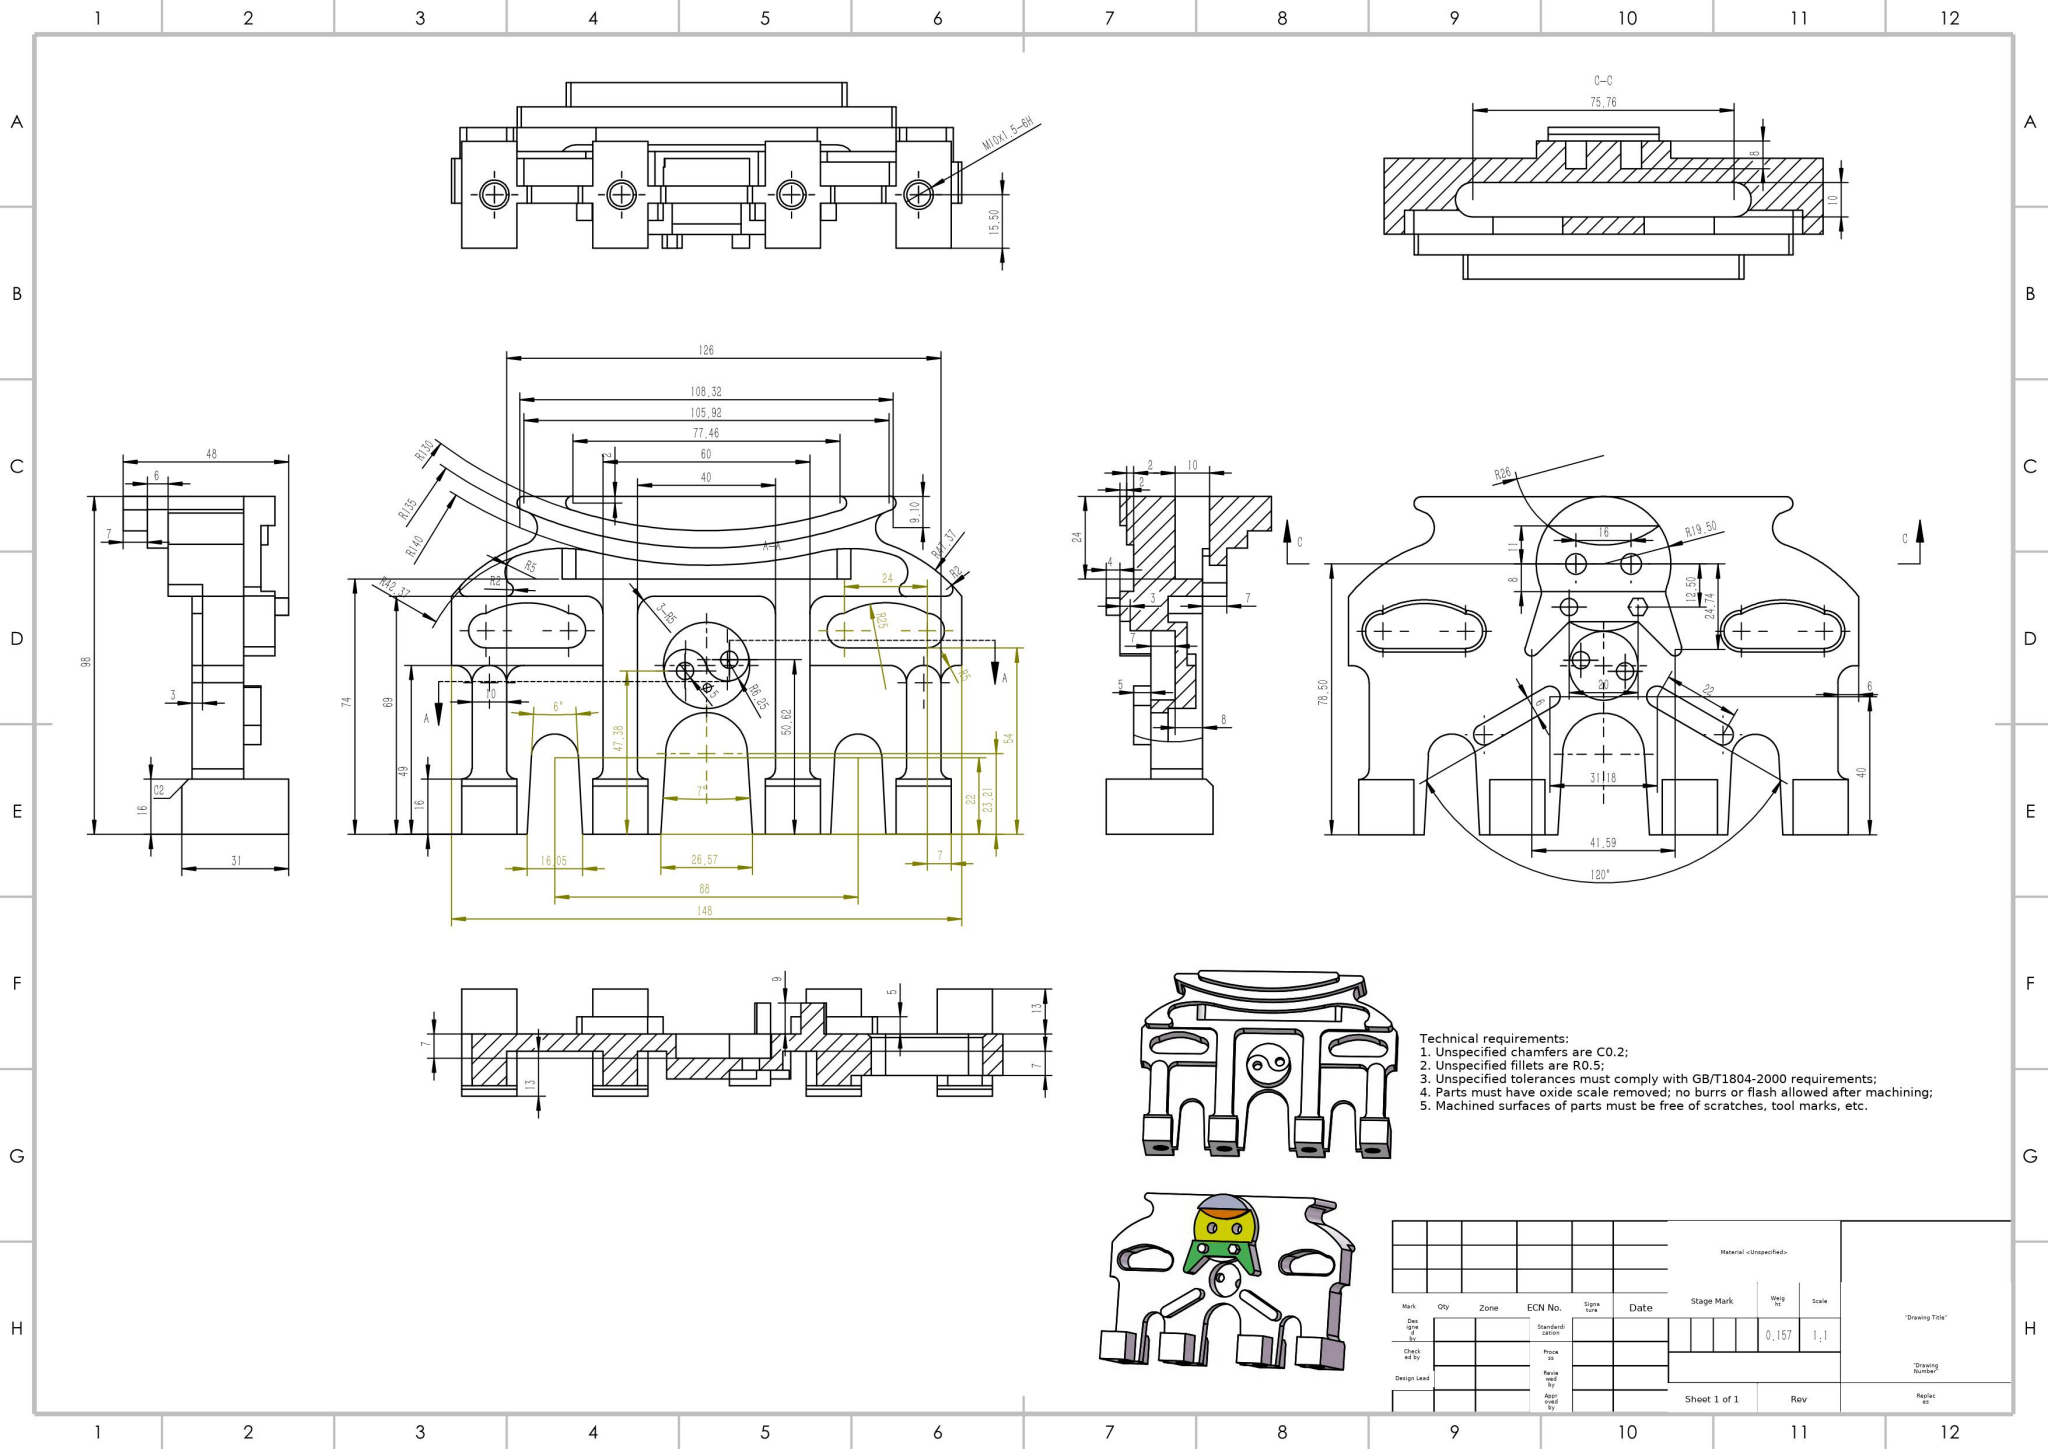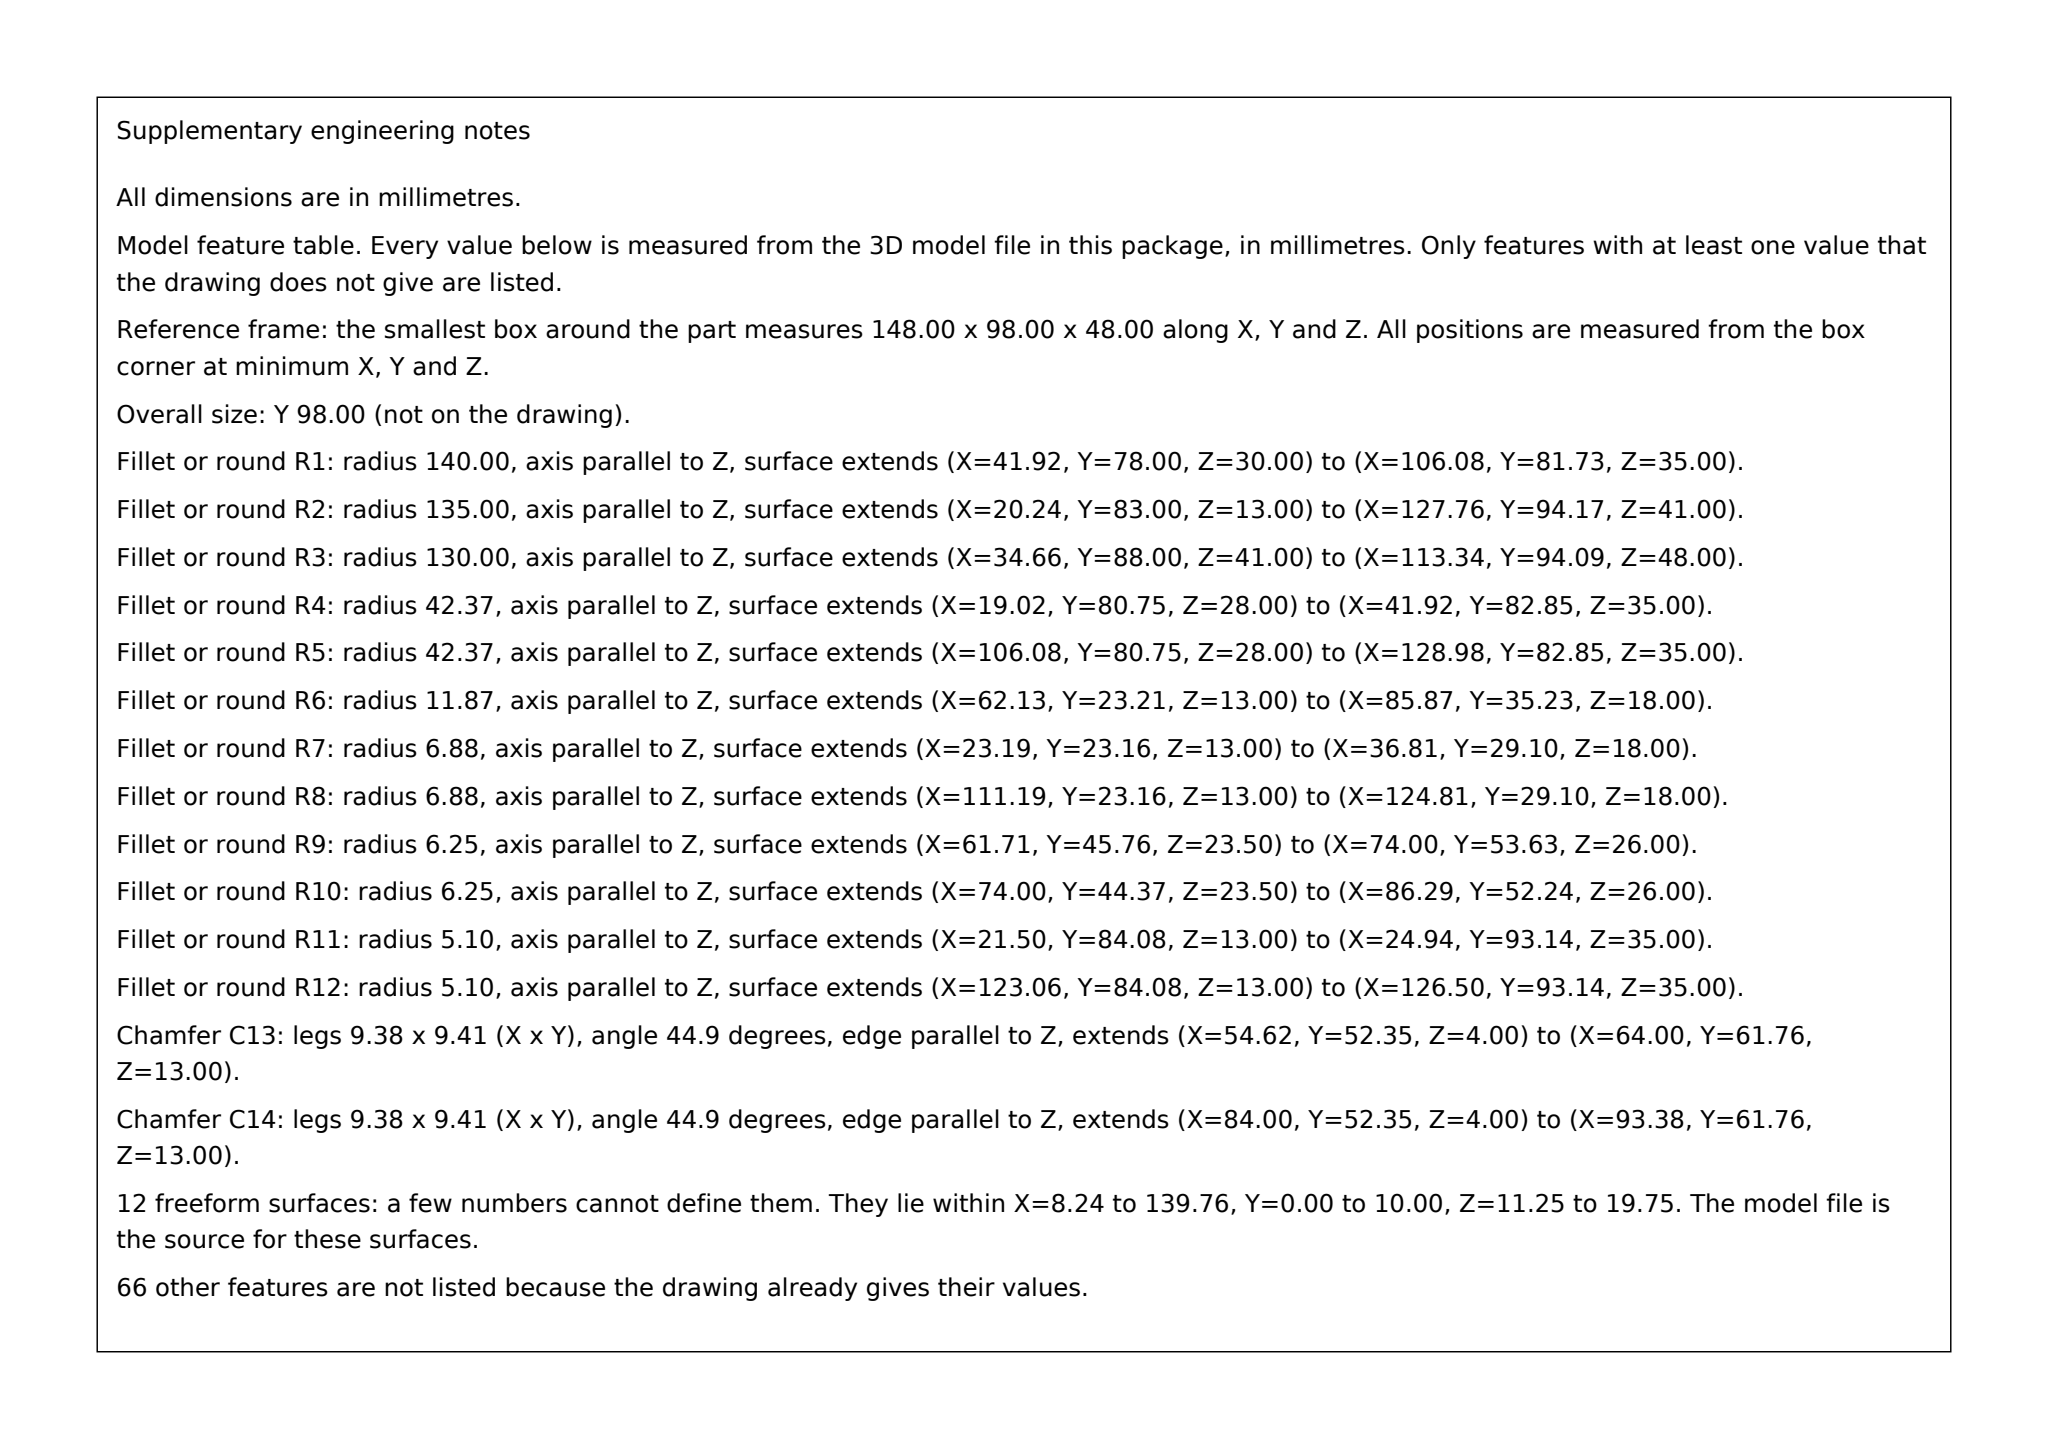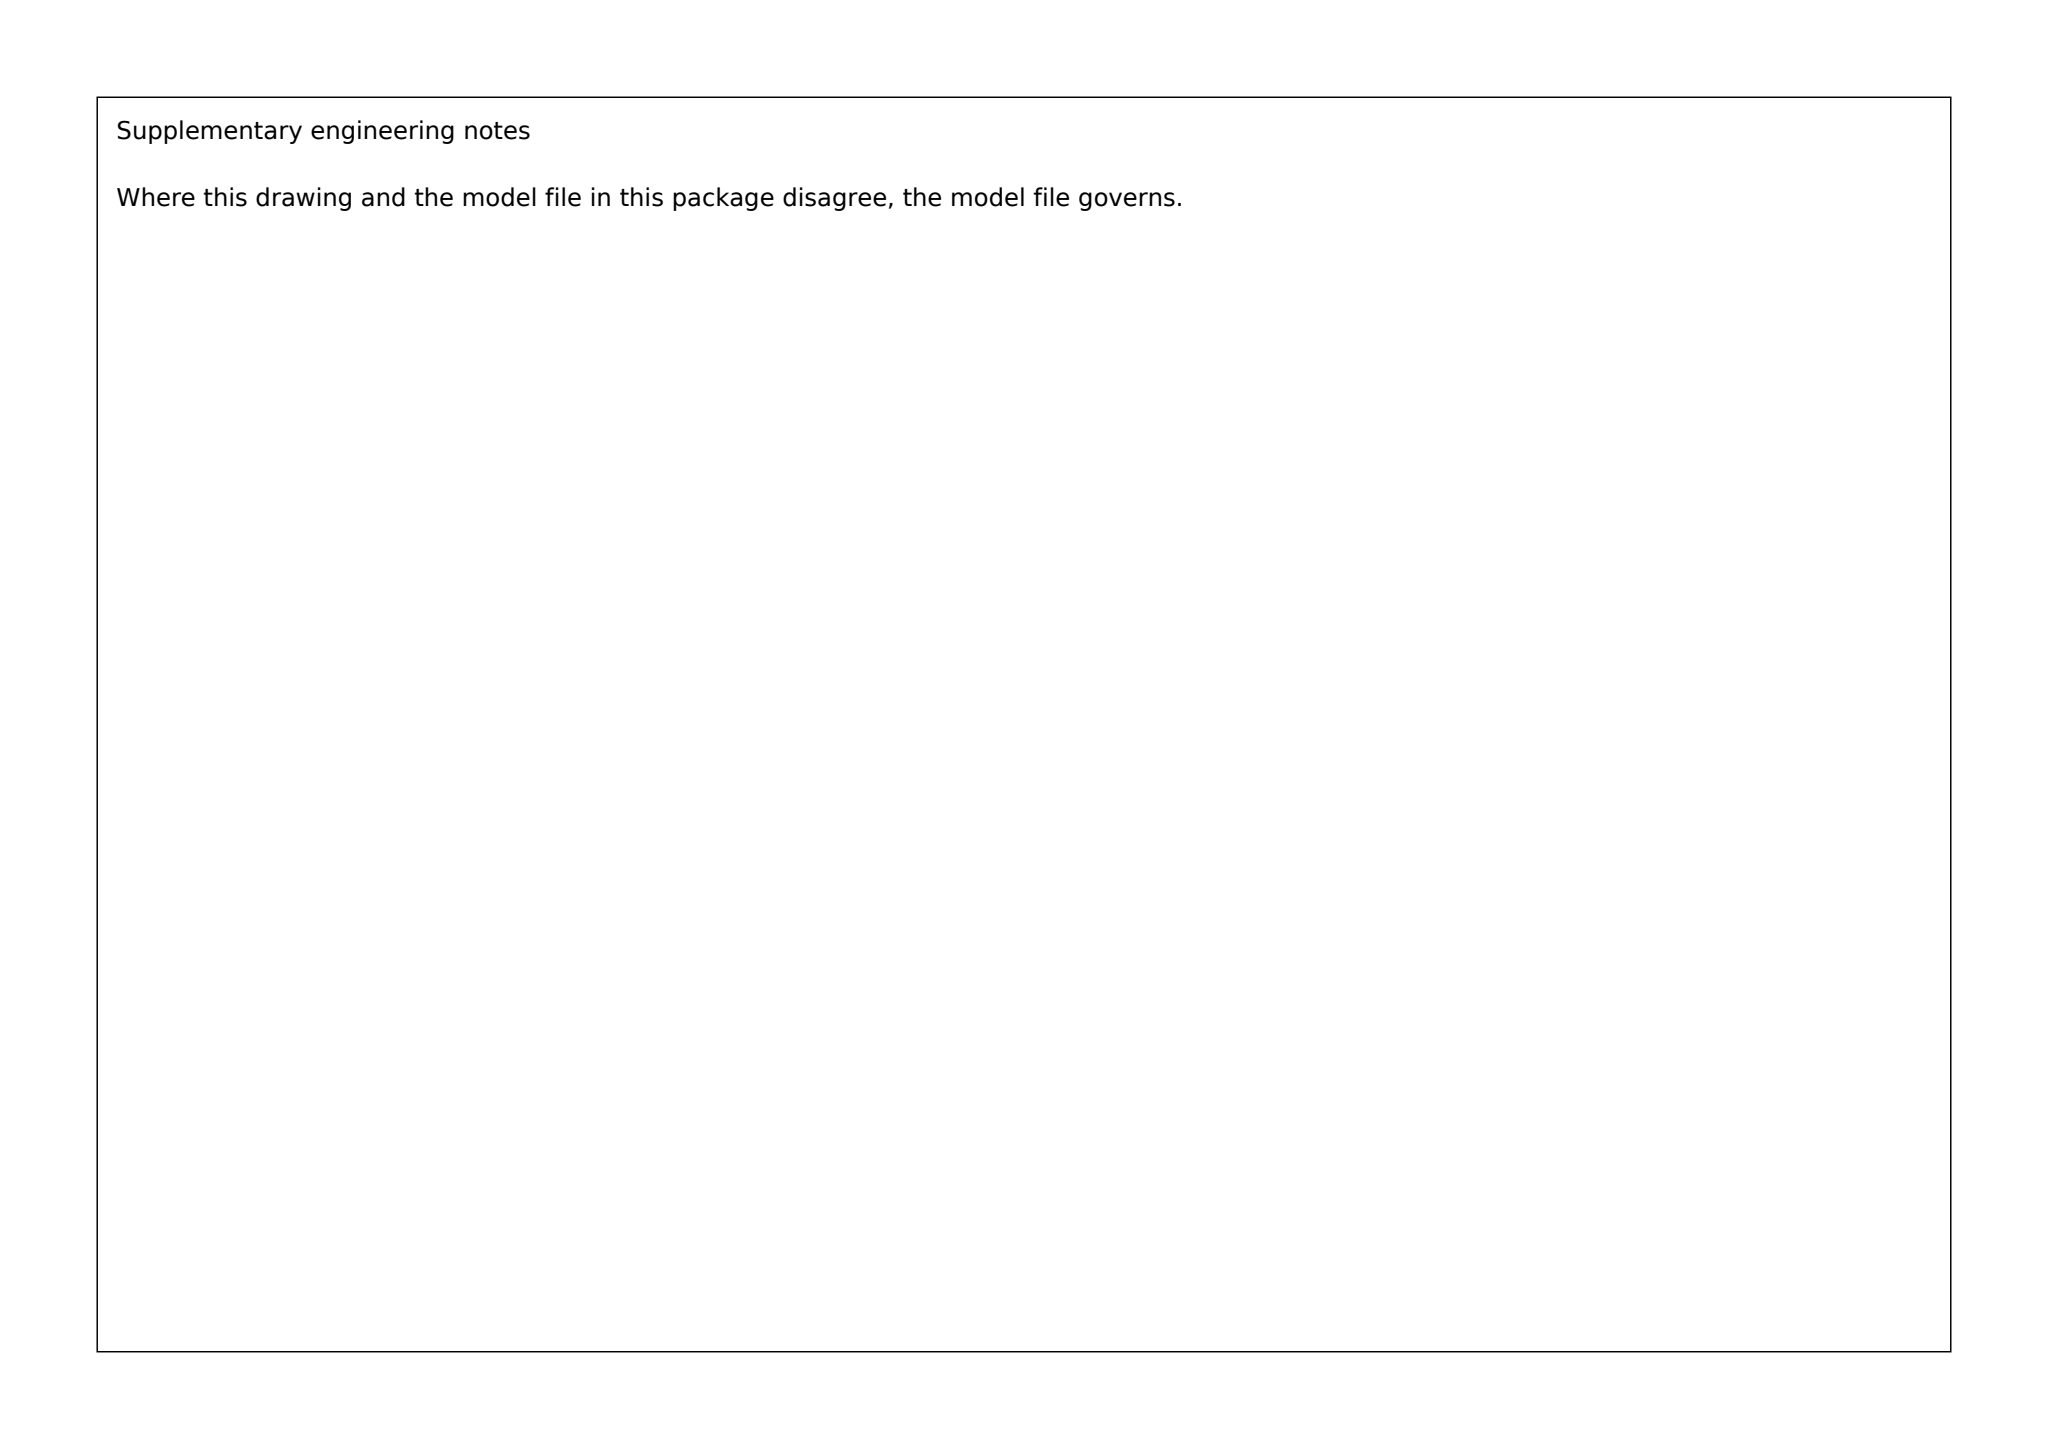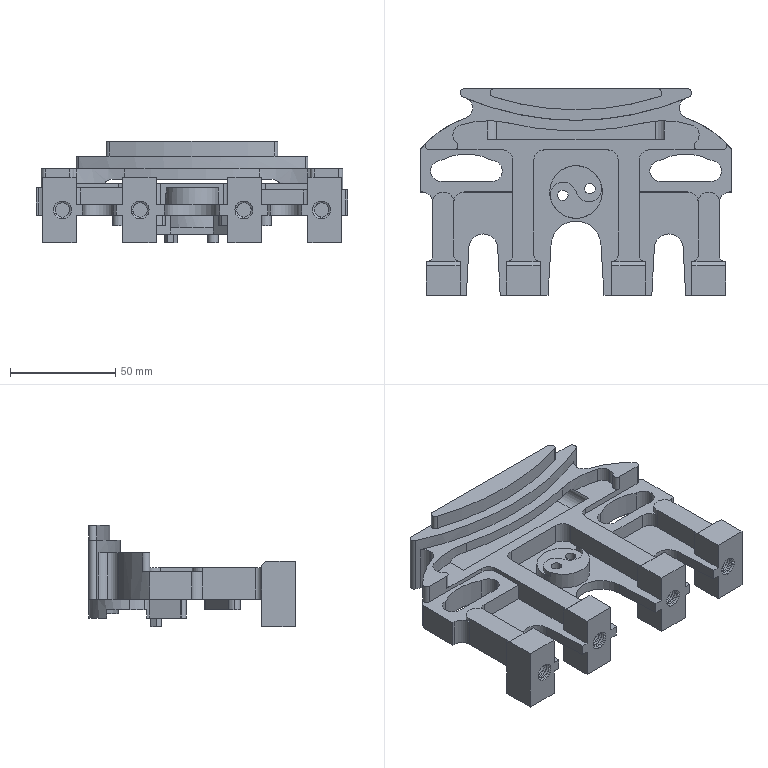Part | SolidWorks | mm | 1 solid | 288 faces | box 148 x 98 x 48 mm | volume 157179 mm3 | cylinder 148 | plane 120 | spline 12 | cone 8 | commonest cylinder face diameters 8.5 x56 10 x21 6 x18 4 x15 5 x6 39 x4 12.5 x3 10.2 x3